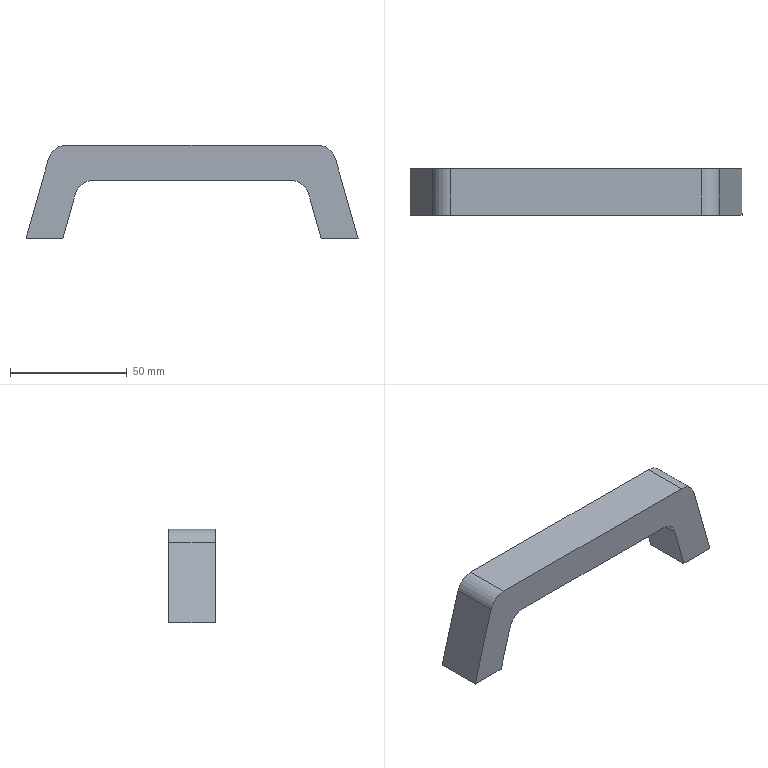Component | SolidWorks | 1UnitDrawer-1_DrawerPanelHandle-1 | 1 solid | 20 faces | box 142 x 20 x 40 mm | volume 52496 mm3 | plane 12 | cylinder 8 | commonest cylinder face diameters 6.5 x4 16 x4
build123d program:
from build123d import *

# Parameters (mm, degrees)
EXTRUDE1_DEPTH = 20
SKETCH2_R      = 3.25
EXTRUDE2_DEPTH = 5


with BuildPart() as part:
    # Sketch1 → Extrude1 (new body)
    with BuildSketch(Plane.XY):
        with BuildLine():
            Line((-20, 71), (14.169, 61.375))
            ThreePointArc((14.169, 61.375), (18.378, 58.504), (20, 53.675))
            Line((20, 53.675), (20, -53.675))
            ThreePointArc((20, -53.675), (18.378, -58.504), (14.169, -61.375))
            Line((14.169, -61.375), (-20, -71))
            Line((-20, -71), (-20, -55.279))
            Line((-20, -55.279), (-0.8309, -49.879))
            ThreePointArc((-0.8309, -49.879), (3.378, -47.008), (5, -42.179))
            Line((5, -42.179), (5, 42.179))
            ThreePointArc((5, 42.179), (3.378, 47.008), (-0.8309, 49.879))
            Line((-0.8309, 49.879), (-20, 55.279))
            Line((-20, 55.279), (-20, 71))
        make_face()
    extrude(amount=EXTRUDE1_DEPTH)

    # Sketch2 → Extrude2 (cut)
    with BuildSketch(Plane.ZY.offset(20)):
        with Locations((10, 65.015)):
            Circle(SKETCH2_R)
        with Locations((10, -65.015)):
            Circle(SKETCH2_R)
    extrude(amount=-EXTRUDE2_DEPTH, mode=Mode.SUBTRACT)


solid = part.part

# Placed as in the assembly
solid = solid.moved(Location((-1806.445, -724.443, 440), (90, 0, 90)))
STEP:
#1=CARTESIAN_POINT('',(-68.56,-28.787,16.732));
#2=VERTEX_POINT('',#1);
#3=CARTESIAN_POINT('',(-68.56,-29.043,16.732));
#4=VERTEX_POINT('',#3);
#5=CARTESIAN_POINT('',(-68.56,-28.915,16.732));
#6=DIRECTION('',(0.,-0.,-1.));
#7=DIRECTION('',(0.,-1.,0.));
#8=AXIS2_PLACEMENT_3D('',#5,#6,#7);
#9=CIRCLE('',#8,0.128);
#10=EDGE_CURVE('',#2,#4,#9,.T.);
#11=ORIENTED_EDGE('',*,*,#10,.F.);
#12=CARTESIAN_POINT('',(-68.56,-28.787,16.535));
#13=VERTEX_POINT('',#12);
#14=CARTESIAN_POINT('',(-68.56,-28.787,16.732));
#15=DIRECTION('',(0.,-0.,-1.));
#16=VECTOR('',#15,39.37);
#17=LINE('',#14,#16);
#18=EDGE_CURVE('',#2,#13,#17,.T.);
#19=ORIENTED_EDGE('',*,*,#18,.T.);
#20=CARTESIAN_POINT('',(-68.56,-29.043,16.535));
#21=VERTEX_POINT('',#20);
#22=CARTESIAN_POINT('',(-68.56,-28.915,16.535));
#23=DIRECTION('',(0.,-0.,-1.));
#24=DIRECTION('',(0.,-1.,0.));
#25=AXIS2_PLACEMENT_3D('',#22,#23,#24);
#26=CIRCLE('',#25,0.128);
#27=EDGE_CURVE('',#13,#21,#26,.T.);
#28=ORIENTED_EDGE('',*,*,#27,.T.);
#29=CARTESIAN_POINT('',(-68.56,-29.043,16.732));
#30=DIRECTION('',(0.,-0.,-1.));
#31=VECTOR('',#30,39.37);
#32=LINE('',#29,#31);
#33=EDGE_CURVE('',#4,#21,#32,.T.);
#34=ORIENTED_EDGE('',*,*,#33,.F.);
#35=EDGE_LOOP('',(#11,#19,#28,#34));
#36=FACE_OUTER_BOUND('',#35,.T.);
#37=CARTESIAN_POINT('',(-68.56,-28.915,16.732));
#38=DIRECTION('',(0.,-0.,-1.));
#39=DIRECTION('',(0.,-1.,0.));
#40=AXIS2_PLACEMENT_3D('',#37,#38,#39);
#41=CYLINDRICAL_SURFACE('',#40,0.128);
#42=ADVANCED_FACE('',(#36),#41,.F.);
#43=CARTESIAN_POINT('',(-73.68,-28.787,16.732));
#44=VERTEX_POINT('',#43);
#45=CARTESIAN_POINT('',(-73.68,-29.043,16.732));
#46=VERTEX_POINT('',#45);
#47=CARTESIAN_POINT('',(-73.68,-28.915,16.732));
#48=DIRECTION('',(0.,-0.,-1.));
#49=DIRECTION('',(0.,-1.,0.));
#50=AXIS2_PLACEMENT_3D('',#47,#48,#49);
#51=CIRCLE('',#50,0.128);
#52=EDGE_CURVE('',#44,#46,#51,.T.);
#53=ORIENTED_EDGE('',*,*,#52,.F.);
#54=CARTESIAN_POINT('',(-73.68,-28.787,16.535));
#55=VERTEX_POINT('',#54);
#56=CARTESIAN_POINT('',(-73.68,-28.787,16.732));
#57=DIRECTION('',(0.,-0.,-1.));
#58=VECTOR('',#57,39.37);
#59=LINE('',#56,#58);
#60=EDGE_CURVE('',#44,#55,#59,.T.);
#61=ORIENTED_EDGE('',*,*,#60,.T.);
#62=CARTESIAN_POINT('',(-73.68,-29.043,16.535));
#63=VERTEX_POINT('',#62);
#64=CARTESIAN_POINT('',(-73.68,-28.915,16.535));
#65=DIRECTION('',(0.,-0.,-1.));
#66=DIRECTION('',(0.,-1.,0.));
#67=AXIS2_PLACEMENT_3D('',#64,#65,#66);
#68=CIRCLE('',#67,0.128);
#69=EDGE_CURVE('',#55,#63,#68,.T.);
#70=ORIENTED_EDGE('',*,*,#69,.T.);
#71=CARTESIAN_POINT('',(-73.68,-29.043,16.732));
#72=DIRECTION('',(0.,-0.,-1.));
#73=VECTOR('',#72,39.37);
#74=LINE('',#71,#73);
#75=EDGE_CURVE('',#46,#63,#74,.T.);
#76=ORIENTED_EDGE('',*,*,#75,.F.);
#77=EDGE_LOOP('',(#53,#61,#70,#76));
#78=FACE_OUTER_BOUND('',#77,.T.);
#79=CARTESIAN_POINT('',(-73.68,-28.915,16.732));
#80=DIRECTION('',(0.,-0.,-1.));
#81=DIRECTION('',(0.,-1.,0.));
#82=AXIS2_PLACEMENT_3D('',#79,#80,#81);
#83=CYLINDRICAL_SURFACE('',#82,0.128);
#84=ADVANCED_FACE('',(#78),#83,.F.);
#85=CARTESIAN_POINT('',(-68.325,-28.521,16.535));
#86=VERTEX_POINT('',#85);
#87=CARTESIAN_POINT('',(-68.704,-28.521,17.881));
#88=VERTEX_POINT('',#87);
#89=CARTESIAN_POINT('',(-68.325,-28.521,16.535));
#90=DIRECTION('',(-0.2711,0.,0.9625));
#91=VECTOR('',#90,39.37);
#92=LINE('',#89,#91);
#93=EDGE_CURVE('',#86,#88,#92,.T.);
#94=ORIENTED_EDGE('',*,*,#93,.T.);
#95=CARTESIAN_POINT('',(-68.704,-29.309,17.881));
#96=VERTEX_POINT('',#95);
#97=CARTESIAN_POINT('',(-68.704,-29.309,17.881));
#98=DIRECTION('',(-0.,1.,-0.));
#99=VECTOR('',#98,39.37);
#100=LINE('',#97,#99);
#101=EDGE_CURVE('',#96,#88,#100,.T.);
#102=ORIENTED_EDGE('',*,*,#101,.F.);
#103=CARTESIAN_POINT('',(-68.325,-29.309,16.535));
#104=VERTEX_POINT('',#103);
#105=CARTESIAN_POINT('',(-68.325,-29.309,16.535));
#106=DIRECTION('',(-0.2711,0.,0.9625));
#107=VECTOR('',#106,39.37);
#108=LINE('',#105,#107);
#109=EDGE_CURVE('',#104,#96,#108,.T.);
#110=ORIENTED_EDGE('',*,*,#109,.F.);
#111=CARTESIAN_POINT('',(-68.325,-29.309,16.535));
#112=DIRECTION('',(-0.,1.,-0.));
#113=VECTOR('',#112,39.37);
#114=LINE('',#111,#113);
#115=EDGE_CURVE('',#104,#86,#114,.T.);
#116=ORIENTED_EDGE('',*,*,#115,.T.);
#117=EDGE_LOOP('',(#94,#102,#110,#116));
#118=FACE_OUTER_BOUND('',#117,.T.);
#119=CARTESIAN_POINT('',(-68.325,-29.309,16.535));
#120=DIRECTION('',(-0.9625,-0.,-0.2711));
#121=DIRECTION('',(0.2711,-0.,-0.9625));
#122=AXIS2_PLACEMENT_3D('',#119,#120,#121);
#123=PLANE('',#122);
#124=ADVANCED_FACE('',(#118),#123,.F.);
#125=CARTESIAN_POINT('',(-69.007,-28.521,18.11));
#126=VERTEX_POINT('',#125);
#127=CARTESIAN_POINT('',(-69.007,-28.521,17.795));
#128=DIRECTION('',(0.,-1.,0.));
#129=DIRECTION('',(0.,0.,1.));
#130=AXIS2_PLACEMENT_3D('',#127,#128,#129);
#131=CIRCLE('',#130,0.315);
#132=EDGE_CURVE('',#88,#126,#131,.T.);
#133=ORIENTED_EDGE('',*,*,#132,.T.);
#134=CARTESIAN_POINT('',(-69.007,-29.309,18.11));
#135=VERTEX_POINT('',#134);
#136=CARTESIAN_POINT('',(-69.007,-29.309,18.11));
#137=DIRECTION('',(-0.,1.,-0.));
#138=VECTOR('',#137,39.37);
#139=LINE('',#136,#138);
#140=EDGE_CURVE('',#135,#126,#139,.T.);
#141=ORIENTED_EDGE('',*,*,#140,.F.);
#142=CARTESIAN_POINT('',(-69.007,-29.309,17.795));
#143=DIRECTION('',(0.,-1.,0.));
#144=DIRECTION('',(0.,0.,1.));
#145=AXIS2_PLACEMENT_3D('',#142,#143,#144);
#146=CIRCLE('',#145,0.315);
#147=EDGE_CURVE('',#96,#135,#146,.T.);
#148=ORIENTED_EDGE('',*,*,#147,.F.);
#149=ORIENTED_EDGE('',*,*,#101,.T.);
#150=EDGE_LOOP('',(#133,#141,#148,#149));
#151=FACE_OUTER_BOUND('',#150,.T.);
#152=CARTESIAN_POINT('',(-69.007,-29.309,17.795));
#153=DIRECTION('',(-0.,1.,-0.));
#154=DIRECTION('',(0.,-0.,-1.));
#155=AXIS2_PLACEMENT_3D('',#152,#153,#154);
#156=CYLINDRICAL_SURFACE('',#155,0.315);
#157=ADVANCED_FACE('',(#151),#156,.T.);
#158=CARTESIAN_POINT('',(-73.233,-28.521,18.11));
#159=VERTEX_POINT('',#158);
#160=CARTESIAN_POINT('',(-69.007,-28.521,18.11));
#161=DIRECTION('',(-1.,-0.,-0.));
#162=VECTOR('',#161,39.37);
#163=LINE('',#160,#162);
#164=EDGE_CURVE('',#126,#159,#163,.T.);
#165=ORIENTED_EDGE('',*,*,#164,.T.);
#166=CARTESIAN_POINT('',(-73.233,-29.309,18.11));
#167=VERTEX_POINT('',#166);
#168=CARTESIAN_POINT('',(-73.233,-29.309,18.11));
#169=DIRECTION('',(-0.,1.,-0.));
#170=VECTOR('',#169,39.37);
#171=LINE('',#168,#170);
#172=EDGE_CURVE('',#167,#159,#171,.T.);
#173=ORIENTED_EDGE('',*,*,#172,.F.);
#174=CARTESIAN_POINT('',(-69.007,-29.309,18.11));
#175=DIRECTION('',(-1.,-0.,-0.));
#176=VECTOR('',#175,39.37);
#177=LINE('',#174,#176);
#178=EDGE_CURVE('',#135,#167,#177,.T.);
#179=ORIENTED_EDGE('',*,*,#178,.F.);
#180=ORIENTED_EDGE('',*,*,#140,.T.);
#181=EDGE_LOOP('',(#165,#173,#179,#180));
#182=FACE_OUTER_BOUND('',#181,.T.);
#183=CARTESIAN_POINT('',(-69.007,-29.309,18.11));
#184=DIRECTION('',(0.,-0.,-1.));
#185=DIRECTION('',(1.,0.,0.));
#186=AXIS2_PLACEMENT_3D('',#183,#184,#185);
#187=PLANE('',#186);
#188=ADVANCED_FACE('',(#182),#187,.F.);
#189=CARTESIAN_POINT('',(-73.536,-28.521,17.881));
#190=VERTEX_POINT('',#189);
#191=CARTESIAN_POINT('',(-73.233,-28.521,17.795));
#192=DIRECTION('',(0.,-1.,0.));
#193=DIRECTION('',(0.,0.,1.));
#194=AXIS2_PLACEMENT_3D('',#191,#192,#193);
#195=CIRCLE('',#194,0.315);
#196=EDGE_CURVE('',#159,#190,#195,.T.);
#197=ORIENTED_EDGE('',*,*,#196,.T.);
#198=CARTESIAN_POINT('',(-73.536,-29.309,17.881));
#199=VERTEX_POINT('',#198);
#200=CARTESIAN_POINT('',(-73.536,-29.309,17.881));
#201=DIRECTION('',(-0.,1.,-0.));
#202=VECTOR('',#201,39.37);
#203=LINE('',#200,#202);
#204=EDGE_CURVE('',#199,#190,#203,.T.);
#205=ORIENTED_EDGE('',*,*,#204,.F.);
#206=CARTESIAN_POINT('',(-73.233,-29.309,17.795));
#207=DIRECTION('',(0.,-1.,0.));
#208=DIRECTION('',(0.,0.,1.));
#209=AXIS2_PLACEMENT_3D('',#206,#207,#208);
#210=CIRCLE('',#209,0.315);
#211=EDGE_CURVE('',#167,#199,#210,.T.);
#212=ORIENTED_EDGE('',*,*,#211,.F.);
#213=ORIENTED_EDGE('',*,*,#172,.T.);
#214=EDGE_LOOP('',(#197,#205,#212,#213));
#215=FACE_OUTER_BOUND('',#214,.T.);
#216=CARTESIAN_POINT('',(-73.233,-29.309,17.795));
#217=DIRECTION('',(-0.,1.,-0.));
#218=DIRECTION('',(0.,-0.,-1.));
#219=AXIS2_PLACEMENT_3D('',#216,#217,#218);
#220=CYLINDRICAL_SURFACE('',#219,0.315);
#221=ADVANCED_FACE('',(#215),#220,.T.);
#222=CARTESIAN_POINT('',(-73.915,-28.521,16.535));
#223=VERTEX_POINT('',#222);
#224=CARTESIAN_POINT('',(-73.915,-28.521,16.535));
#225=DIRECTION('',(-0.2711,-0.,-0.9625));
#226=VECTOR('',#225,39.37);
#227=LINE('',#224,#226);
#228=EDGE_CURVE('',#190,#223,#227,.T.);
#229=ORIENTED_EDGE('',*,*,#228,.T.);
#230=CARTESIAN_POINT('',(-73.915,-29.309,16.535));
#231=VERTEX_POINT('',#230);
#232=CARTESIAN_POINT('',(-73.915,-29.309,16.535));
#233=DIRECTION('',(-0.,1.,-0.));
#234=VECTOR('',#233,39.37);
#235=LINE('',#232,#234);
#236=EDGE_CURVE('',#231,#223,#235,.T.);
#237=ORIENTED_EDGE('',*,*,#236,.F.);
#238=CARTESIAN_POINT('',(-73.915,-29.309,16.535));
#239=DIRECTION('',(-0.2711,-0.,-0.9625));
#240=VECTOR('',#239,39.37);
#241=LINE('',#238,#240);
#242=EDGE_CURVE('',#199,#231,#241,.T.);
#243=ORIENTED_EDGE('',*,*,#242,.F.);
#244=ORIENTED_EDGE('',*,*,#204,.T.);
#245=EDGE_LOOP('',(#229,#237,#243,#244));
#246=FACE_OUTER_BOUND('',#245,.T.);
#247=CARTESIAN_POINT('',(-73.915,-29.309,16.535));
#248=DIRECTION('',(0.9625,0.,-0.2711));
#249=DIRECTION('',(0.2711,0.,0.9625));
#250=AXIS2_PLACEMENT_3D('',#247,#248,#249);
#251=PLANE('',#250);
#252=ADVANCED_FACE('',(#246),#251,.F.);
#253=CARTESIAN_POINT('',(-73.68,-28.915,16.535));
#254=DIRECTION('',(0.,-0.,-1.));
#255=DIRECTION('',(0.,-1.,0.));
#256=AXIS2_PLACEMENT_3D('',#253,#254,#255);
#257=CIRCLE('',#256,0.128);
#258=EDGE_CURVE('',#63,#55,#257,.T.);
#259=ORIENTED_EDGE('',*,*,#258,.F.);
#260=ORIENTED_EDGE('',*,*,#69,.F.);
#261=EDGE_LOOP('',(#259,#260));
#262=FACE_BOUND('',#261,.T.);
#263=CARTESIAN_POINT('',(-73.296,-28.521,16.535));
#264=VERTEX_POINT('',#263);
#265=CARTESIAN_POINT('',(-73.296,-28.521,16.535));
#266=DIRECTION('',(1.,0.,0.));
#267=VECTOR('',#266,39.37);
#268=LINE('',#265,#267);
#269=EDGE_CURVE('',#223,#264,#268,.T.);
#270=ORIENTED_EDGE('',*,*,#269,.T.);
#271=CARTESIAN_POINT('',(-73.296,-29.309,16.535));
#272=VERTEX_POINT('',#271);
#273=CARTESIAN_POINT('',(-73.296,-29.309,16.535));
#274=DIRECTION('',(-0.,1.,-0.));
#275=VECTOR('',#274,39.37);
#276=LINE('',#273,#275);
#277=EDGE_CURVE('',#272,#264,#276,.T.);
#278=ORIENTED_EDGE('',*,*,#277,.F.);
#279=CARTESIAN_POINT('',(-73.296,-29.309,16.535));
#280=DIRECTION('',(1.,0.,0.));
#281=VECTOR('',#280,39.37);
#282=LINE('',#279,#281);
#283=EDGE_CURVE('',#231,#272,#282,.T.);
#284=ORIENTED_EDGE('',*,*,#283,.F.);
#285=ORIENTED_EDGE('',*,*,#236,.T.);
#286=EDGE_LOOP('',(#270,#278,#284,#285));
#287=FACE_OUTER_BOUND('',#286,.T.);
#288=CARTESIAN_POINT('',(-73.296,-29.309,16.535));
#289=DIRECTION('',(-0.,0.,1.));
#290=DIRECTION('',(-0.,1.,-0.));
#291=AXIS2_PLACEMENT_3D('',#288,#289,#290);
#292=PLANE('',#291);
#293=ADVANCED_FACE('',(#262,#287),#292,.F.);
#294=CARTESIAN_POINT('',(-73.084,-28.521,17.29));
#295=VERTEX_POINT('',#294);
#296=CARTESIAN_POINT('',(-73.296,-28.521,16.535));
#297=DIRECTION('',(0.2711,0.,0.9625));
#298=VECTOR('',#297,39.37);
#299=LINE('',#296,#298);
#300=EDGE_CURVE('',#264,#295,#299,.T.);
#301=ORIENTED_EDGE('',*,*,#300,.T.);
#302=CARTESIAN_POINT('',(-73.084,-29.309,17.29));
#303=VERTEX_POINT('',#302);
#304=CARTESIAN_POINT('',(-73.084,-29.309,17.29));
#305=DIRECTION('',(-0.,1.,-0.));
#306=VECTOR('',#305,39.37);
#307=LINE('',#304,#306);
#308=EDGE_CURVE('',#303,#295,#307,.T.);
#309=ORIENTED_EDGE('',*,*,#308,.F.);
#310=CARTESIAN_POINT('',(-73.296,-29.309,16.535));
#311=DIRECTION('',(0.2711,0.,0.9625));
#312=VECTOR('',#311,39.37);
#313=LINE('',#310,#312);
#314=EDGE_CURVE('',#272,#303,#313,.T.);
#315=ORIENTED_EDGE('',*,*,#314,.F.);
#316=ORIENTED_EDGE('',*,*,#277,.T.);
#317=EDGE_LOOP('',(#301,#309,#315,#316));
#318=FACE_OUTER_BOUND('',#317,.T.);
#319=CARTESIAN_POINT('',(-73.296,-29.309,16.535));
#320=DIRECTION('',(-0.9625,-0.,0.2711));
#321=DIRECTION('',(-0.2711,-0.,-0.9625));
#322=AXIS2_PLACEMENT_3D('',#319,#320,#321);
#323=PLANE('',#322);
#324=ADVANCED_FACE('',(#318),#323,.F.);
#325=CARTESIAN_POINT('',(-72.78,-28.521,17.52));
#326=VERTEX_POINT('',#325);
#327=CARTESIAN_POINT('',(-72.78,-28.521,17.205));
#328=DIRECTION('',(-0.,1.,-0.));
#329=DIRECTION('',(0.,0.,1.));
#330=AXIS2_PLACEMENT_3D('',#327,#328,#329);
#331=CIRCLE('',#330,0.315);
#332=EDGE_CURVE('',#295,#326,#331,.T.);
#333=ORIENTED_EDGE('',*,*,#332,.T.);
#334=CARTESIAN_POINT('',(-72.78,-29.309,17.52));
#335=VERTEX_POINT('',#334);
#336=CARTESIAN_POINT('',(-72.78,-29.309,17.52));
#337=DIRECTION('',(-0.,1.,-0.));
#338=VECTOR('',#337,39.37);
#339=LINE('',#336,#338);
#340=EDGE_CURVE('',#335,#326,#339,.T.);
#341=ORIENTED_EDGE('',*,*,#340,.F.);
#342=CARTESIAN_POINT('',(-72.78,-29.309,17.205));
#343=DIRECTION('',(-0.,1.,-0.));
#344=DIRECTION('',(0.,0.,1.));
#345=AXIS2_PLACEMENT_3D('',#342,#343,#344);
#346=CIRCLE('',#345,0.315);
#347=EDGE_CURVE('',#303,#335,#346,.T.);
#348=ORIENTED_EDGE('',*,*,#347,.F.);
#349=ORIENTED_EDGE('',*,*,#308,.T.);
#350=EDGE_LOOP('',(#333,#341,#348,#349));
#351=FACE_OUTER_BOUND('',#350,.T.);
#352=CARTESIAN_POINT('',(-72.78,-29.309,17.205));
#353=DIRECTION('',(-0.,1.,-0.));
#354=DIRECTION('',(0.,-0.,-1.));
#355=AXIS2_PLACEMENT_3D('',#352,#353,#354);
#356=CYLINDRICAL_SURFACE('',#355,0.315);
#357=ADVANCED_FACE('',(#351),#356,.F.);
#358=CARTESIAN_POINT('',(-69.459,-28.521,17.52));
#359=VERTEX_POINT('',#358);
#360=CARTESIAN_POINT('',(-72.78,-28.521,17.52));
#361=DIRECTION('',(1.,0.,0.));
#362=VECTOR('',#361,39.37);
#363=LINE('',#360,#362);
#364=EDGE_CURVE('',#326,#359,#363,.T.);
#365=ORIENTED_EDGE('',*,*,#364,.T.);
#366=CARTESIAN_POINT('',(-69.459,-29.309,17.52));
#367=VERTEX_POINT('',#366);
#368=CARTESIAN_POINT('',(-69.459,-29.309,17.52));
#369=DIRECTION('',(-0.,1.,-0.));
#370=VECTOR('',#369,39.37);
#371=LINE('',#368,#370);
#372=EDGE_CURVE('',#367,#359,#371,.T.);
#373=ORIENTED_EDGE('',*,*,#372,.F.);
#374=CARTESIAN_POINT('',(-72.78,-29.309,17.52));
#375=DIRECTION('',(1.,0.,0.));
#376=VECTOR('',#375,39.37);
#377=LINE('',#374,#376);
#378=EDGE_CURVE('',#335,#367,#377,.T.);
#379=ORIENTED_EDGE('',*,*,#378,.F.);
#380=ORIENTED_EDGE('',*,*,#340,.T.);
#381=EDGE_LOOP('',(#365,#373,#379,#380));
#382=FACE_OUTER_BOUND('',#381,.T.);
#383=CARTESIAN_POINT('',(-72.78,-29.309,17.52));
#384=DIRECTION('',(-0.,0.,1.));
#385=DIRECTION('',(-1.,-0.,-0.));
#386=AXIS2_PLACEMENT_3D('',#383,#384,#385);
#387=PLANE('',#386);
#388=ADVANCED_FACE('',(#382),#387,.F.);
#389=CARTESIAN_POINT('',(-69.156,-28.521,17.29));
#390=VERTEX_POINT('',#389);
#391=CARTESIAN_POINT('',(-69.459,-28.521,17.205));
#392=DIRECTION('',(-0.,1.,-0.));
#393=DIRECTION('',(0.,-0.,-1.));
#394=AXIS2_PLACEMENT_3D('',#391,#392,#393);
#395=CIRCLE('',#394,0.315);
#396=EDGE_CURVE('',#359,#390,#395,.T.);
#397=ORIENTED_EDGE('',*,*,#396,.T.);
#398=CARTESIAN_POINT('',(-69.156,-29.309,17.29));
#399=VERTEX_POINT('',#398);
#400=CARTESIAN_POINT('',(-69.156,-29.309,17.29));
#401=DIRECTION('',(-0.,1.,-0.));
#402=VECTOR('',#401,39.37);
#403=LINE('',#400,#402);
#404=EDGE_CURVE('',#399,#390,#403,.T.);
#405=ORIENTED_EDGE('',*,*,#404,.F.);
#406=CARTESIAN_POINT('',(-69.459,-29.309,17.205));
#407=DIRECTION('',(-0.,1.,-0.));
#408=DIRECTION('',(0.,-0.,-1.));
#409=AXIS2_PLACEMENT_3D('',#406,#407,#408);
#410=CIRCLE('',#409,0.315);
#411=EDGE_CURVE('',#367,#399,#410,.T.);
#412=ORIENTED_EDGE('',*,*,#411,.F.);
#413=ORIENTED_EDGE('',*,*,#372,.T.);
#414=EDGE_LOOP('',(#397,#405,#412,#413));
#415=FACE_OUTER_BOUND('',#414,.T.);
#416=CARTESIAN_POINT('',(-69.459,-29.309,17.205));
#417=DIRECTION('',(-0.,1.,-0.));
#418=DIRECTION('',(0.,-0.,-1.));
#419=AXIS2_PLACEMENT_3D('',#416,#417,#418);
#420=CYLINDRICAL_SURFACE('',#419,0.315);
#421=ADVANCED_FACE('',(#415),#420,.F.);
#422=CARTESIAN_POINT('',(-68.944,-28.521,16.535));
#423=VERTEX_POINT('',#422);
#424=CARTESIAN_POINT('',(-68.944,-28.521,16.535));
#425=DIRECTION('',(0.2711,-0.,-0.9625));
#426=VECTOR('',#425,39.37);
#427=LINE('',#424,#426);
#428=EDGE_CURVE('',#390,#423,#427,.T.);
#429=ORIENTED_EDGE('',*,*,#428,.T.);
#430=CARTESIAN_POINT('',(-68.944,-29.309,16.535));
#431=VERTEX_POINT('',#430);
#432=CARTESIAN_POINT('',(-68.944,-29.309,16.535));
#433=DIRECTION('',(-0.,1.,-0.));
#434=VECTOR('',#433,39.37);
#435=LINE('',#432,#434);
#436=EDGE_CURVE('',#431,#423,#435,.T.);
#437=ORIENTED_EDGE('',*,*,#436,.F.);
#438=CARTESIAN_POINT('',(-68.944,-29.309,16.535));
#439=DIRECTION('',(0.2711,-0.,-0.9625));
#440=VECTOR('',#439,39.37);
#441=LINE('',#438,#440);
#442=EDGE_CURVE('',#399,#431,#441,.T.);
#443=ORIENTED_EDGE('',*,*,#442,.F.);
#444=ORIENTED_EDGE('',*,*,#404,.T.);
#445=EDGE_LOOP('',(#429,#437,#443,#444));
#446=FACE_OUTER_BOUND('',#445,.T.);
#447=CARTESIAN_POINT('',(-68.944,-29.309,16.535));
#448=DIRECTION('',(0.9625,0.,0.2711));
#449=DIRECTION('',(-0.2711,0.,0.9625));
#450=AXIS2_PLACEMENT_3D('',#447,#448,#449);
#451=PLANE('',#450);
#452=ADVANCED_FACE('',(#446),#451,.F.);
#453=CARTESIAN_POINT('',(-68.56,-28.915,16.535));
#454=DIRECTION('',(0.,-0.,-1.));
#455=DIRECTION('',(0.,-1.,0.));
#456=AXIS2_PLACEMENT_3D('',#453,#454,#455);
#457=CIRCLE('',#456,0.128);
#458=EDGE_CURVE('',#21,#13,#457,.T.);
#459=ORIENTED_EDGE('',*,*,#458,.F.);
#460=ORIENTED_EDGE('',*,*,#27,.F.);
#461=EDGE_LOOP('',(#459,#460));
#462=FACE_BOUND('',#461,.T.);
#463=CARTESIAN_POINT('',(-68.325,-28.521,16.535));
#464=DIRECTION('',(1.,0.,-0.));
#465=VECTOR('',#464,39.37);
#466=LINE('',#463,#465);
#467=EDGE_CURVE('',#423,#86,#466,.T.);
#468=ORIENTED_EDGE('',*,*,#467,.T.);
#469=ORIENTED_EDGE('',*,*,#115,.F.);
#470=CARTESIAN_POINT('',(-68.325,-29.309,16.535));
#471=DIRECTION('',(1.,0.,-0.));
#472=VECTOR('',#471,39.37);
#473=LINE('',#470,#472);
#474=EDGE_CURVE('',#431,#104,#473,.T.);
#475=ORIENTED_EDGE('',*,*,#474,.F.);
#476=ORIENTED_EDGE('',*,*,#436,.T.);
#477=EDGE_LOOP('',(#468,#469,#475,#476));
#478=FACE_OUTER_BOUND('',#477,.T.);
#479=CARTESIAN_POINT('',(-68.325,-29.309,16.535));
#480=DIRECTION('',(0.,0.,1.));
#481=DIRECTION('',(-1.,-0.,0.));
#482=AXIS2_PLACEMENT_3D('',#479,#480,#481);
#483=PLANE('',#482);
#484=ADVANCED_FACE('',(#462,#478),#483,.F.);
#485=ORIENTED_EDGE('',*,*,#109,.T.);
#486=ORIENTED_EDGE('',*,*,#147,.T.);
#487=ORIENTED_EDGE('',*,*,#178,.T.);
#488=ORIENTED_EDGE('',*,*,#211,.T.);
#489=ORIENTED_EDGE('',*,*,#242,.T.);
#490=ORIENTED_EDGE('',*,*,#283,.T.);
#491=ORIENTED_EDGE('',*,*,#314,.T.);
#492=ORIENTED_EDGE('',*,*,#347,.T.);
#493=ORIENTED_EDGE('',*,*,#378,.T.);
#494=ORIENTED_EDGE('',*,*,#411,.T.);
#495=ORIENTED_EDGE('',*,*,#442,.T.);
#496=ORIENTED_EDGE('',*,*,#474,.T.);
#497=EDGE_LOOP('',(#485,#486,#487,#488,#489,#490,#491,#492,#493,#494,#495,#496));
#498=FACE_OUTER_BOUND('',#497,.T.);
#499=CARTESIAN_POINT('',(-69.007,-29.309,17.795));
#500=DIRECTION('',(0.,-1.,0.));
#501=DIRECTION('',(-0.,0.,1.));
#502=AXIS2_PLACEMENT_3D('',#499,#500,#501);
#503=PLANE('',#502);
#504=ADVANCED_FACE('',(#498),#503,.T.);
#505=ORIENTED_EDGE('',*,*,#93,.F.);
#506=ORIENTED_EDGE('',*,*,#467,.F.);
#507=ORIENTED_EDGE('',*,*,#428,.F.);
#508=ORIENTED_EDGE('',*,*,#396,.F.);
#509=ORIENTED_EDGE('',*,*,#364,.F.);
#510=ORIENTED_EDGE('',*,*,#332,.F.);
#511=ORIENTED_EDGE('',*,*,#300,.F.);
#512=ORIENTED_EDGE('',*,*,#269,.F.);
#513=ORIENTED_EDGE('',*,*,#228,.F.);
#514=ORIENTED_EDGE('',*,*,#196,.F.);
#515=ORIENTED_EDGE('',*,*,#164,.F.);
#516=ORIENTED_EDGE('',*,*,#132,.F.);
#517=EDGE_LOOP('',(#505,#506,#507,#508,#509,#510,#511,#512,#513,#514,#515,#516));
#518=FACE_OUTER_BOUND('',#517,.T.);
#519=CARTESIAN_POINT('',(-69.007,-28.521,17.795));
#520=DIRECTION('',(0.,-1.,0.));
#521=DIRECTION('',(-0.,0.,1.));
#522=AXIS2_PLACEMENT_3D('',#519,#520,#521);
#523=PLANE('',#522);
#524=ADVANCED_FACE('',(#518),#523,.F.);
#525=ORIENTED_EDGE('',*,*,#60,.F.);
#526=CARTESIAN_POINT('',(-73.68,-28.915,16.732));
#527=DIRECTION('',(0.,-0.,-1.));
#528=DIRECTION('',(0.,-1.,0.));
#529=AXIS2_PLACEMENT_3D('',#526,#527,#528);
#530=CIRCLE('',#529,0.128);
#531=EDGE_CURVE('',#46,#44,#530,.T.);
#532=ORIENTED_EDGE('',*,*,#531,.F.);
#533=ORIENTED_EDGE('',*,*,#75,.T.);
#534=ORIENTED_EDGE('',*,*,#258,.T.);
#535=EDGE_LOOP('',(#525,#532,#533,#534));
#536=FACE_OUTER_BOUND('',#535,.T.);
#537=CARTESIAN_POINT('',(-73.68,-28.915,16.732));
#538=DIRECTION('',(0.,-0.,-1.));
#539=DIRECTION('',(0.,-1.,0.));
#540=AXIS2_PLACEMENT_3D('',#537,#538,#539);
#541=CYLINDRICAL_SURFACE('',#540,0.128);
#542=ADVANCED_FACE('',(#536),#541,.F.);
#543=ORIENTED_EDGE('',*,*,#531,.T.);
#544=ORIENTED_EDGE('',*,*,#52,.T.);
#545=EDGE_LOOP('',(#543,#544));
#546=FACE_OUTER_BOUND('',#545,.T.);
#547=CARTESIAN_POINT('',(-73.68,-28.915,16.732));
#548=DIRECTION('',(0.,-0.,-1.));
#549=DIRECTION('',(0.,-1.,0.));
#550=AXIS2_PLACEMENT_3D('',#547,#548,#549);
#551=PLANE('',#550);
#552=ADVANCED_FACE('',(#546),#551,.T.);
#553=ORIENTED_EDGE('',*,*,#18,.F.);
#554=CARTESIAN_POINT('',(-68.56,-28.915,16.732));
#555=DIRECTION('',(0.,-0.,-1.));
#556=DIRECTION('',(0.,-1.,0.));
#557=AXIS2_PLACEMENT_3D('',#554,#555,#556);
#558=CIRCLE('',#557,0.128);
#559=EDGE_CURVE('',#4,#2,#558,.T.);
#560=ORIENTED_EDGE('',*,*,#559,.F.);
#561=ORIENTED_EDGE('',*,*,#33,.T.);
#562=ORIENTED_EDGE('',*,*,#458,.T.);
#563=EDGE_LOOP('',(#553,#560,#561,#562));
#564=FACE_OUTER_BOUND('',#563,.T.);
#565=CARTESIAN_POINT('',(-68.56,-28.915,16.732));
#566=DIRECTION('',(0.,-0.,-1.));
#567=DIRECTION('',(0.,-1.,0.));
#568=AXIS2_PLACEMENT_3D('',#565,#566,#567);
#569=CYLINDRICAL_SURFACE('',#568,0.128);
#570=ADVANCED_FACE('',(#564),#569,.F.);
#571=ORIENTED_EDGE('',*,*,#559,.T.);
#572=ORIENTED_EDGE('',*,*,#10,.T.);
#573=EDGE_LOOP('',(#571,#572));
#574=FACE_OUTER_BOUND('',#573,.T.);
#575=CARTESIAN_POINT('',(-68.56,-28.915,16.732));
#576=DIRECTION('',(0.,-0.,-1.));
#577=DIRECTION('',(0.,-1.,0.));
#578=AXIS2_PLACEMENT_3D('',#575,#576,#577);
#579=PLANE('',#578);
#580=ADVANCED_FACE('',(#574),#579,.T.);
#581=CLOSED_SHELL('',(#42,#84,#124,#157,#188,#221,#252,#293,#324,#357,#388,#421,#452,#484,#504,#524,#542,#552,#570,#580));
#582=MANIFOLD_SOLID_BREP('',#581);
#583=CARTESIAN_POINT('',(0.,0.,0.));
#584=DIRECTION('',(0.,0.,1.));
#585=DIRECTION('',(1.,0.,0.));
#586=AXIS2_PLACEMENT_3D('',#583,#584,#585);
#587=(LENGTH_UNIT()NAMED_UNIT(*)SI_UNIT($,.METRE.));
#588=LENGTH_MEASURE_WITH_UNIT(LENGTH_MEASURE(0.0254),#587);
#589=DIMENSIONAL_EXPONENTS(1.,0.,0.,0.,0.,0.,0.);
#590=(CONVERSION_BASED_UNIT('',#588)LENGTH_UNIT()NAMED_UNIT(#589));
#591=UNCERTAINTY_MEASURE_WITH_UNIT(LENGTH_MEASURE(0.00001),#590,'','');
#592=(NAMED_UNIT(*)PLANE_ANGLE_UNIT()SI_UNIT($,.RADIAN.));
#593=(NAMED_UNIT(*)SI_UNIT($,.STERADIAN.)SOLID_ANGLE_UNIT());
#594=(GEOMETRIC_REPRESENTATION_CONTEXT(3)GLOBAL_UNCERTAINTY_ASSIGNED_CONTEXT((#591))GLOBAL_UNIT_ASSIGNED_CONTEXT((#590,#592,#593))REPRESENTATION_CONTEXT('',''));
#595=ADVANCED_BREP_SHAPE_REPRESENTATION('',(#582,#586),#594);
#596=COLOUR_RGB('',0.7922,0.8196,0.9333);
#597=FILL_AREA_STYLE_COLOUR('',#596);
#598=FILL_AREA_STYLE('',(#597));
#599=SURFACE_STYLE_FILL_AREA(#598);
#600=SURFACE_SIDE_STYLE('',(#599));
#601=SURFACE_STYLE_USAGE(.BOTH.,#600);
#602=PRESENTATION_STYLE_ASSIGNMENT((#601));
#603=STYLED_ITEM('',(#602),#582);
#604=(LENGTH_UNIT()NAMED_UNIT(*)SI_UNIT($,.METRE.));
#605=LENGTH_MEASURE_WITH_UNIT(LENGTH_MEASURE(0.0254),#604);
#606=DIMENSIONAL_EXPONENTS(1.,0.,0.,0.,0.,0.,0.);
#607=(CONVERSION_BASED_UNIT('',#605)LENGTH_UNIT()NAMED_UNIT(#606));
#608=UNCERTAINTY_MEASURE_WITH_UNIT(LENGTH_MEASURE(0.00001),#607,'','');
#609=(NAMED_UNIT(*)PLANE_ANGLE_UNIT()SI_UNIT($,.RADIAN.));
#610=(NAMED_UNIT(*)SI_UNIT($,.STERADIAN.)SOLID_ANGLE_UNIT());
#611=(GEOMETRIC_REPRESENTATION_CONTEXT(3)GLOBAL_UNCERTAINTY_ASSIGNED_CONTEXT((#608))GLOBAL_UNIT_ASSIGNED_CONTEXT((#607,#609,#610))REPRESENTATION_CONTEXT('',''));
#612=MECHANICAL_DESIGN_GEOMETRIC_PRESENTATION_REPRESENTATION('',(#603),#611);
#613=PRESENTATION_LAYER_ASSIGNMENT('','',(#603));